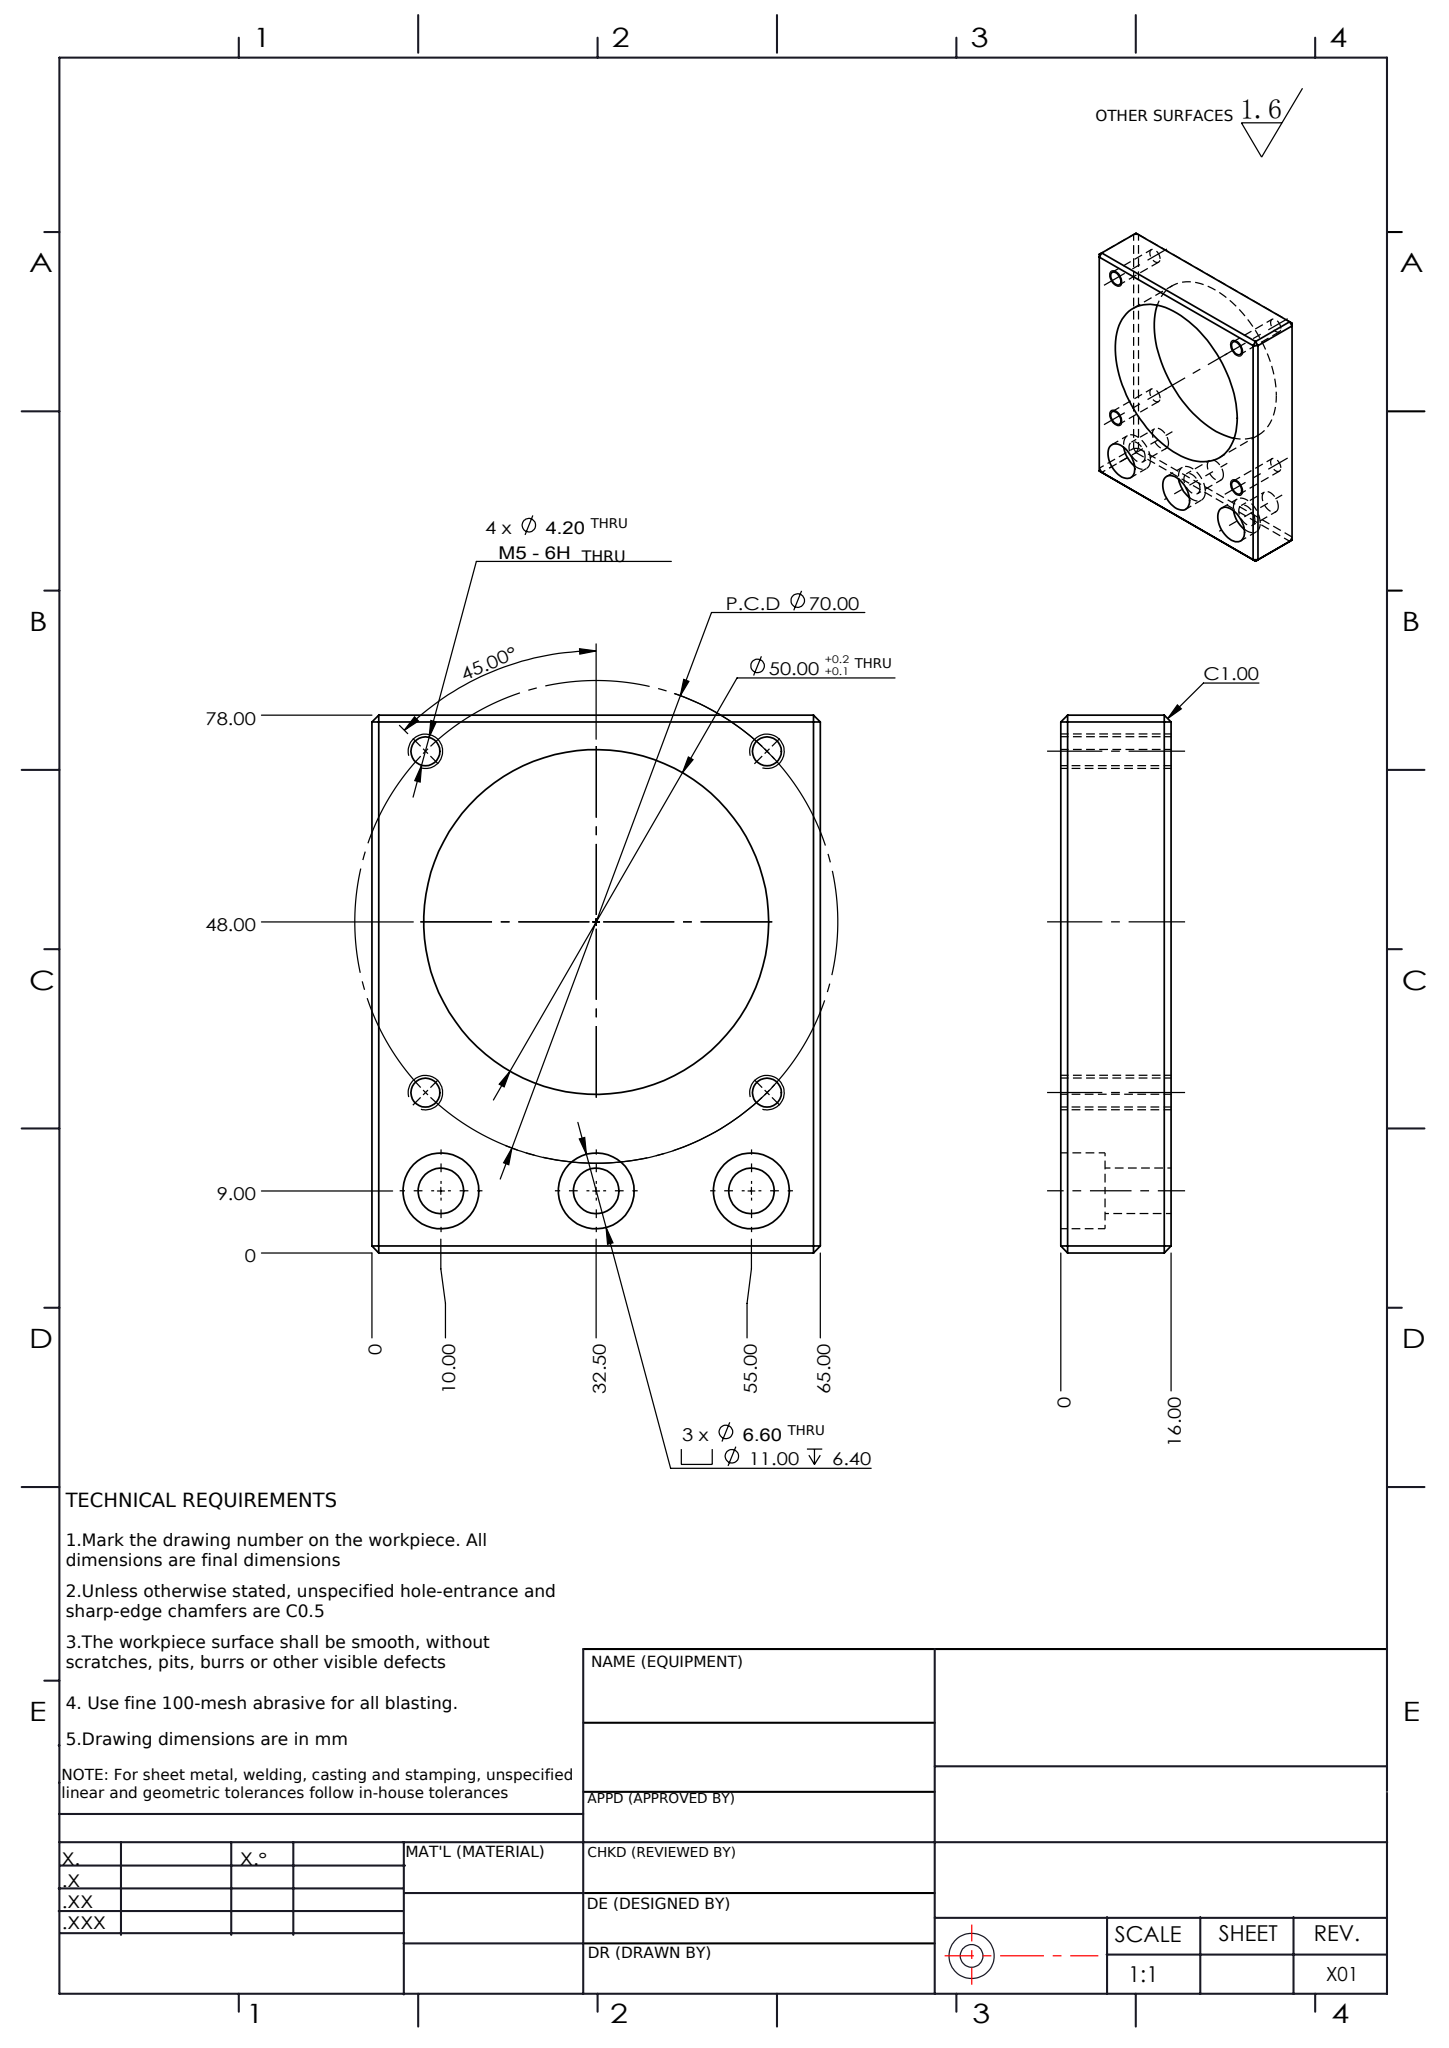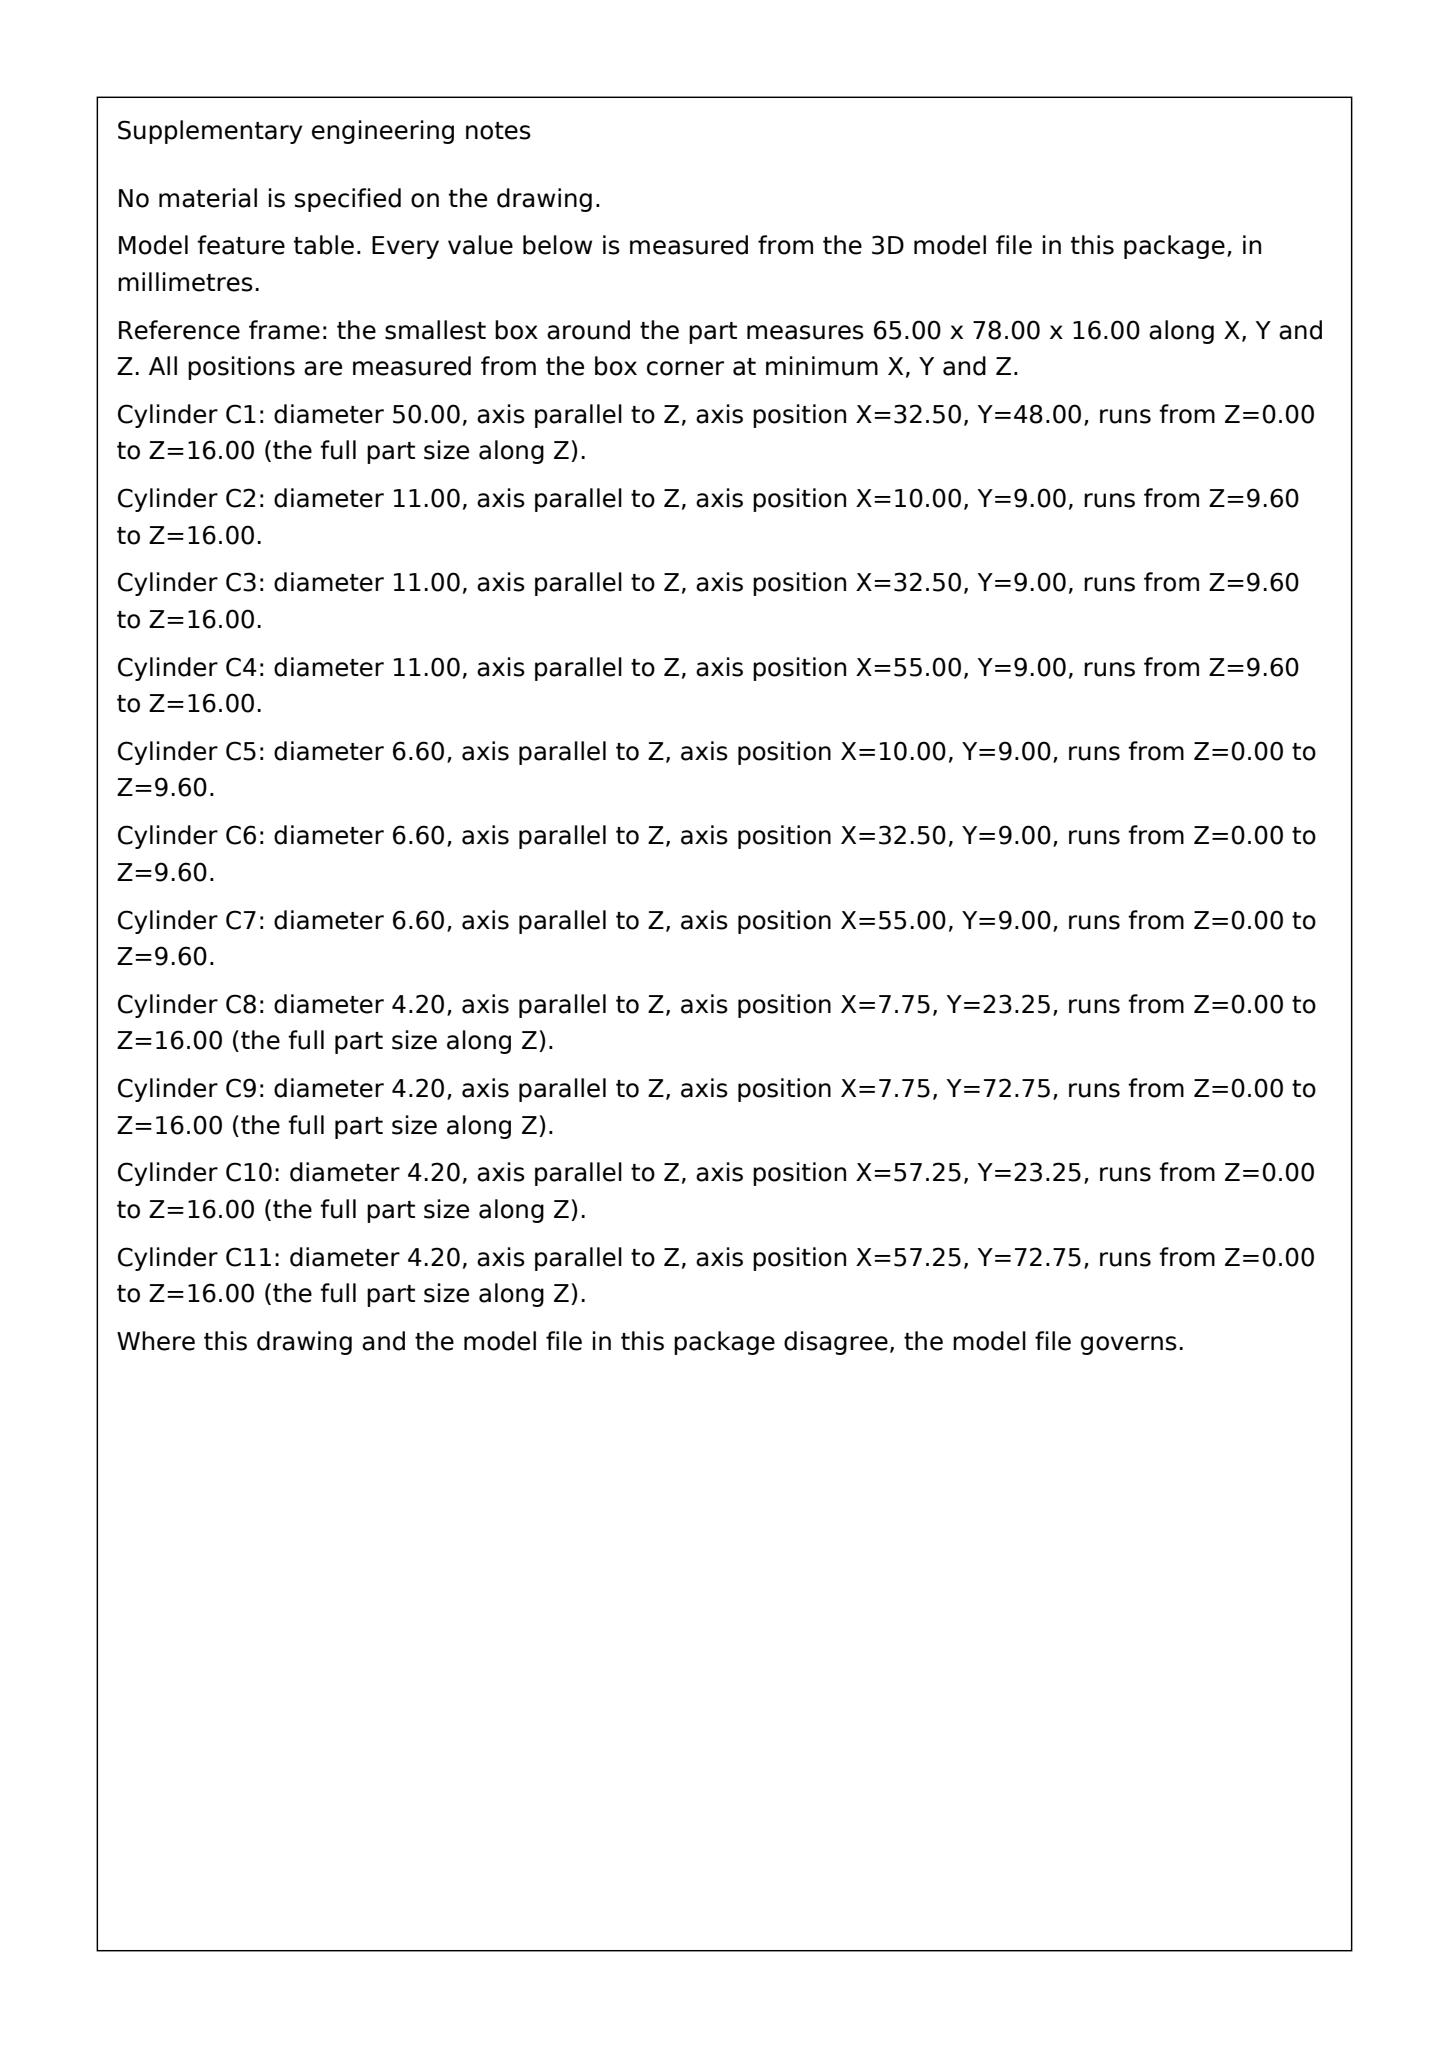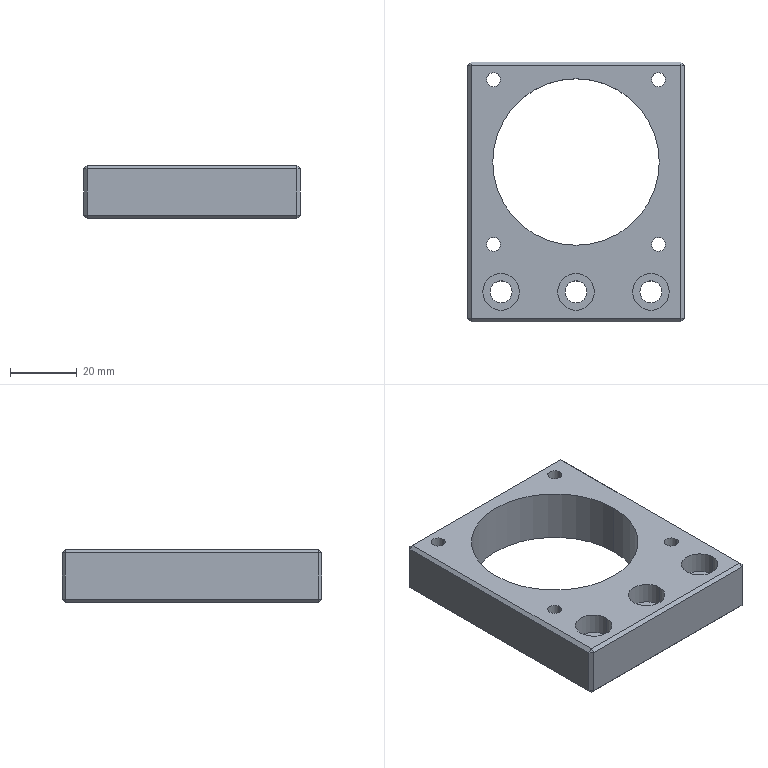Part | SolidWorks | mm | 1 solid | 51 faces | box 65 x 78 x 16 mm | volume 45695 mm3 | plane 29 | cylinder 22 | commonest cylinder face diameters 4.2 x8 11 x6 6.6 x6 50 x2
build123d program:
from build123d import *

# Parameters (mm, degrees)
SKETCH1_W                                       = 65
SKETCH1_H                                       = 78
BOSS_EXTRUDE1_DEPTH                             = 16
SKETCH2_R                                       = 25
CUT_EXTRUDE1_DEPTH                              = 54.228
M5_TAPPED_HOLE1_D                               = 4.2
CHAMFER1_SIZE                                   = 1
M6_HEX_SOCKET_HEAD_CAP_SCREW_CBORE1_D           = 6.6
M6_HEX_SOCKET_HEAD_CAP_SCREW_CBORE1_CBORE_D     = 11
M6_HEX_SOCKET_HEAD_CAP_SCREW_CBORE1_CBORE_DEPTH = 6.4


with BuildPart() as part:
    # Sketch1 → Boss-Extrude1 (new body)
    with BuildSketch(Plane.XY):
        Rectangle(SKETCH1_W, SKETCH1_H)
    extrude(amount=BOSS_EXTRUDE1_DEPTH)

    # Sketch2 → Cut-Extrude1 (cut, through all)
    with BuildSketch(Plane.XY.offset(16)):
        with Locations((0, 9)):
            Circle(SKETCH2_R)
    extrude(amount=-CUT_EXTRUDE1_DEPTH, mode=Mode.SUBTRACT)

    # M5 Tapped Hole1 (through all)
    with Locations(Plane.XY.offset(16)):
        with Locations((-24.75, 33.75), (24.75, 33.75), (24.75, -15.75), (-24.75, -15.75)):
            Hole(M5_TAPPED_HOLE1_D / 2)

    # Chamfer1
    chamfer1_edges = [part.edges().sort_by_distance(p)[0] for p in [
        (-32.5, 0, 16),
        (0, -39, 16),
        (32.5, 0, 16),
        (0, -39, 0),
        (-32.5, 0, 0),
        (0, 39, 0),
        (32.5, 0, 0),
        (0, 39, 16),
        (32.5, -39, 8),
        (-32.5, -39, 8),
        (-32.5, 39, 8),
        (32.5, 39, 8),
    ]]
    chamfer(chamfer1_edges, length=CHAMFER1_SIZE)

    # M6 Hex Socket Head Cap Screw CBORE1 (through all)
    with Locations(Plane.XY.offset(16)):
        with Locations((22.5, -30), (0, -30), (-22.5, -30)):
            CounterBoreHole(M6_HEX_SOCKET_HEAD_CAP_SCREW_CBORE1_D / 2, M6_HEX_SOCKET_HEAD_CAP_SCREW_CBORE1_CBORE_D / 2, M6_HEX_SOCKET_HEAD_CAP_SCREW_CBORE1_CBORE_DEPTH)


solid = part.part